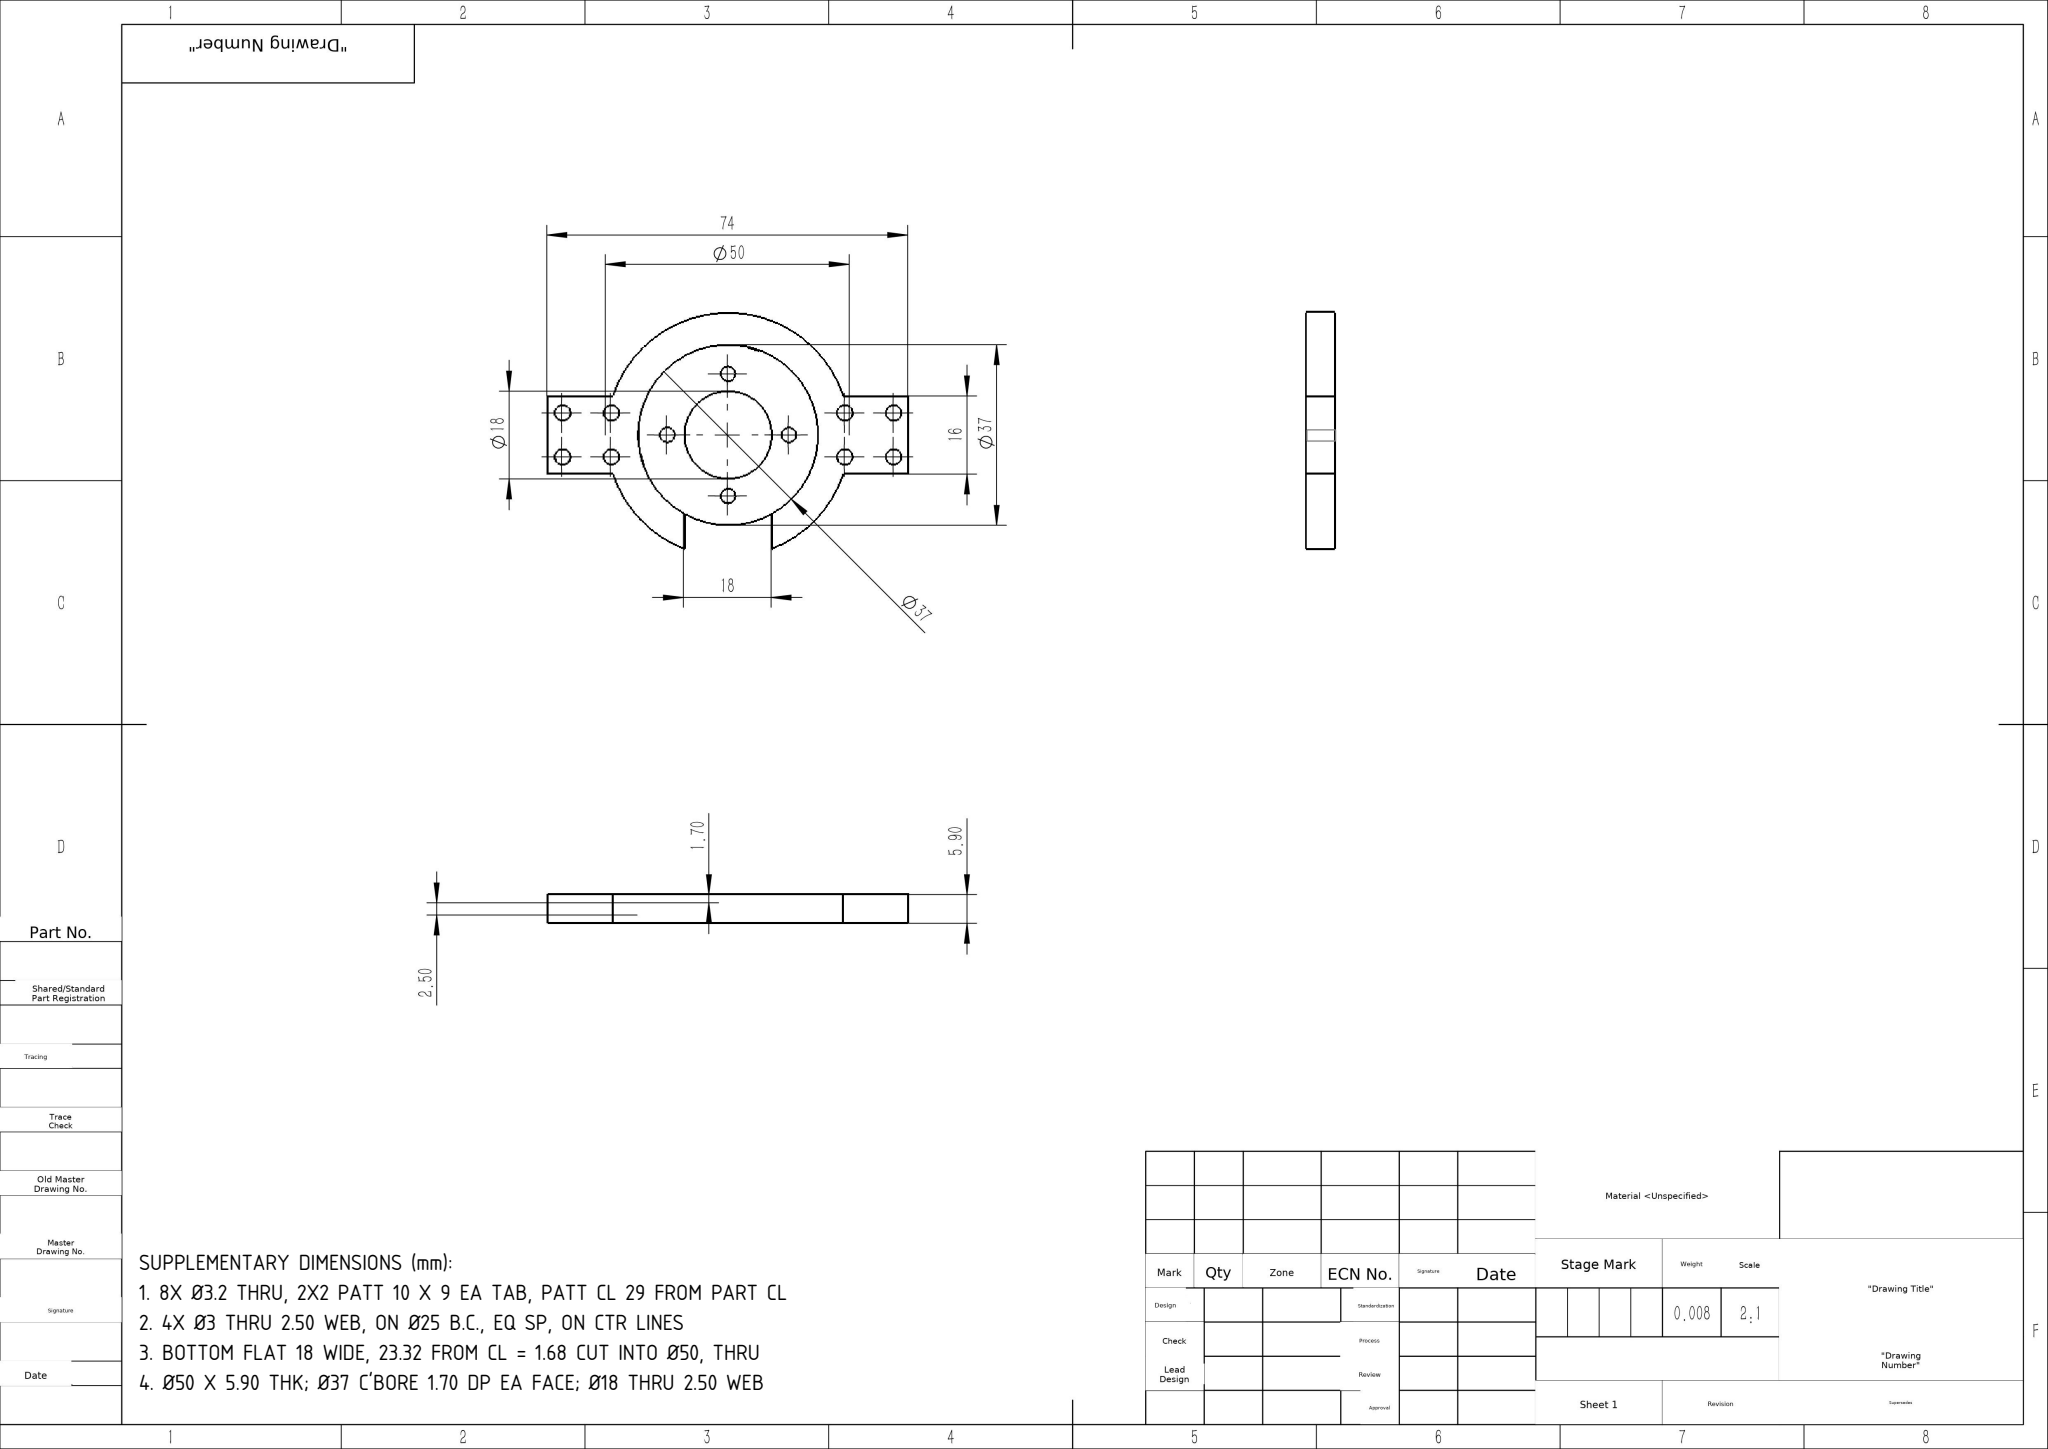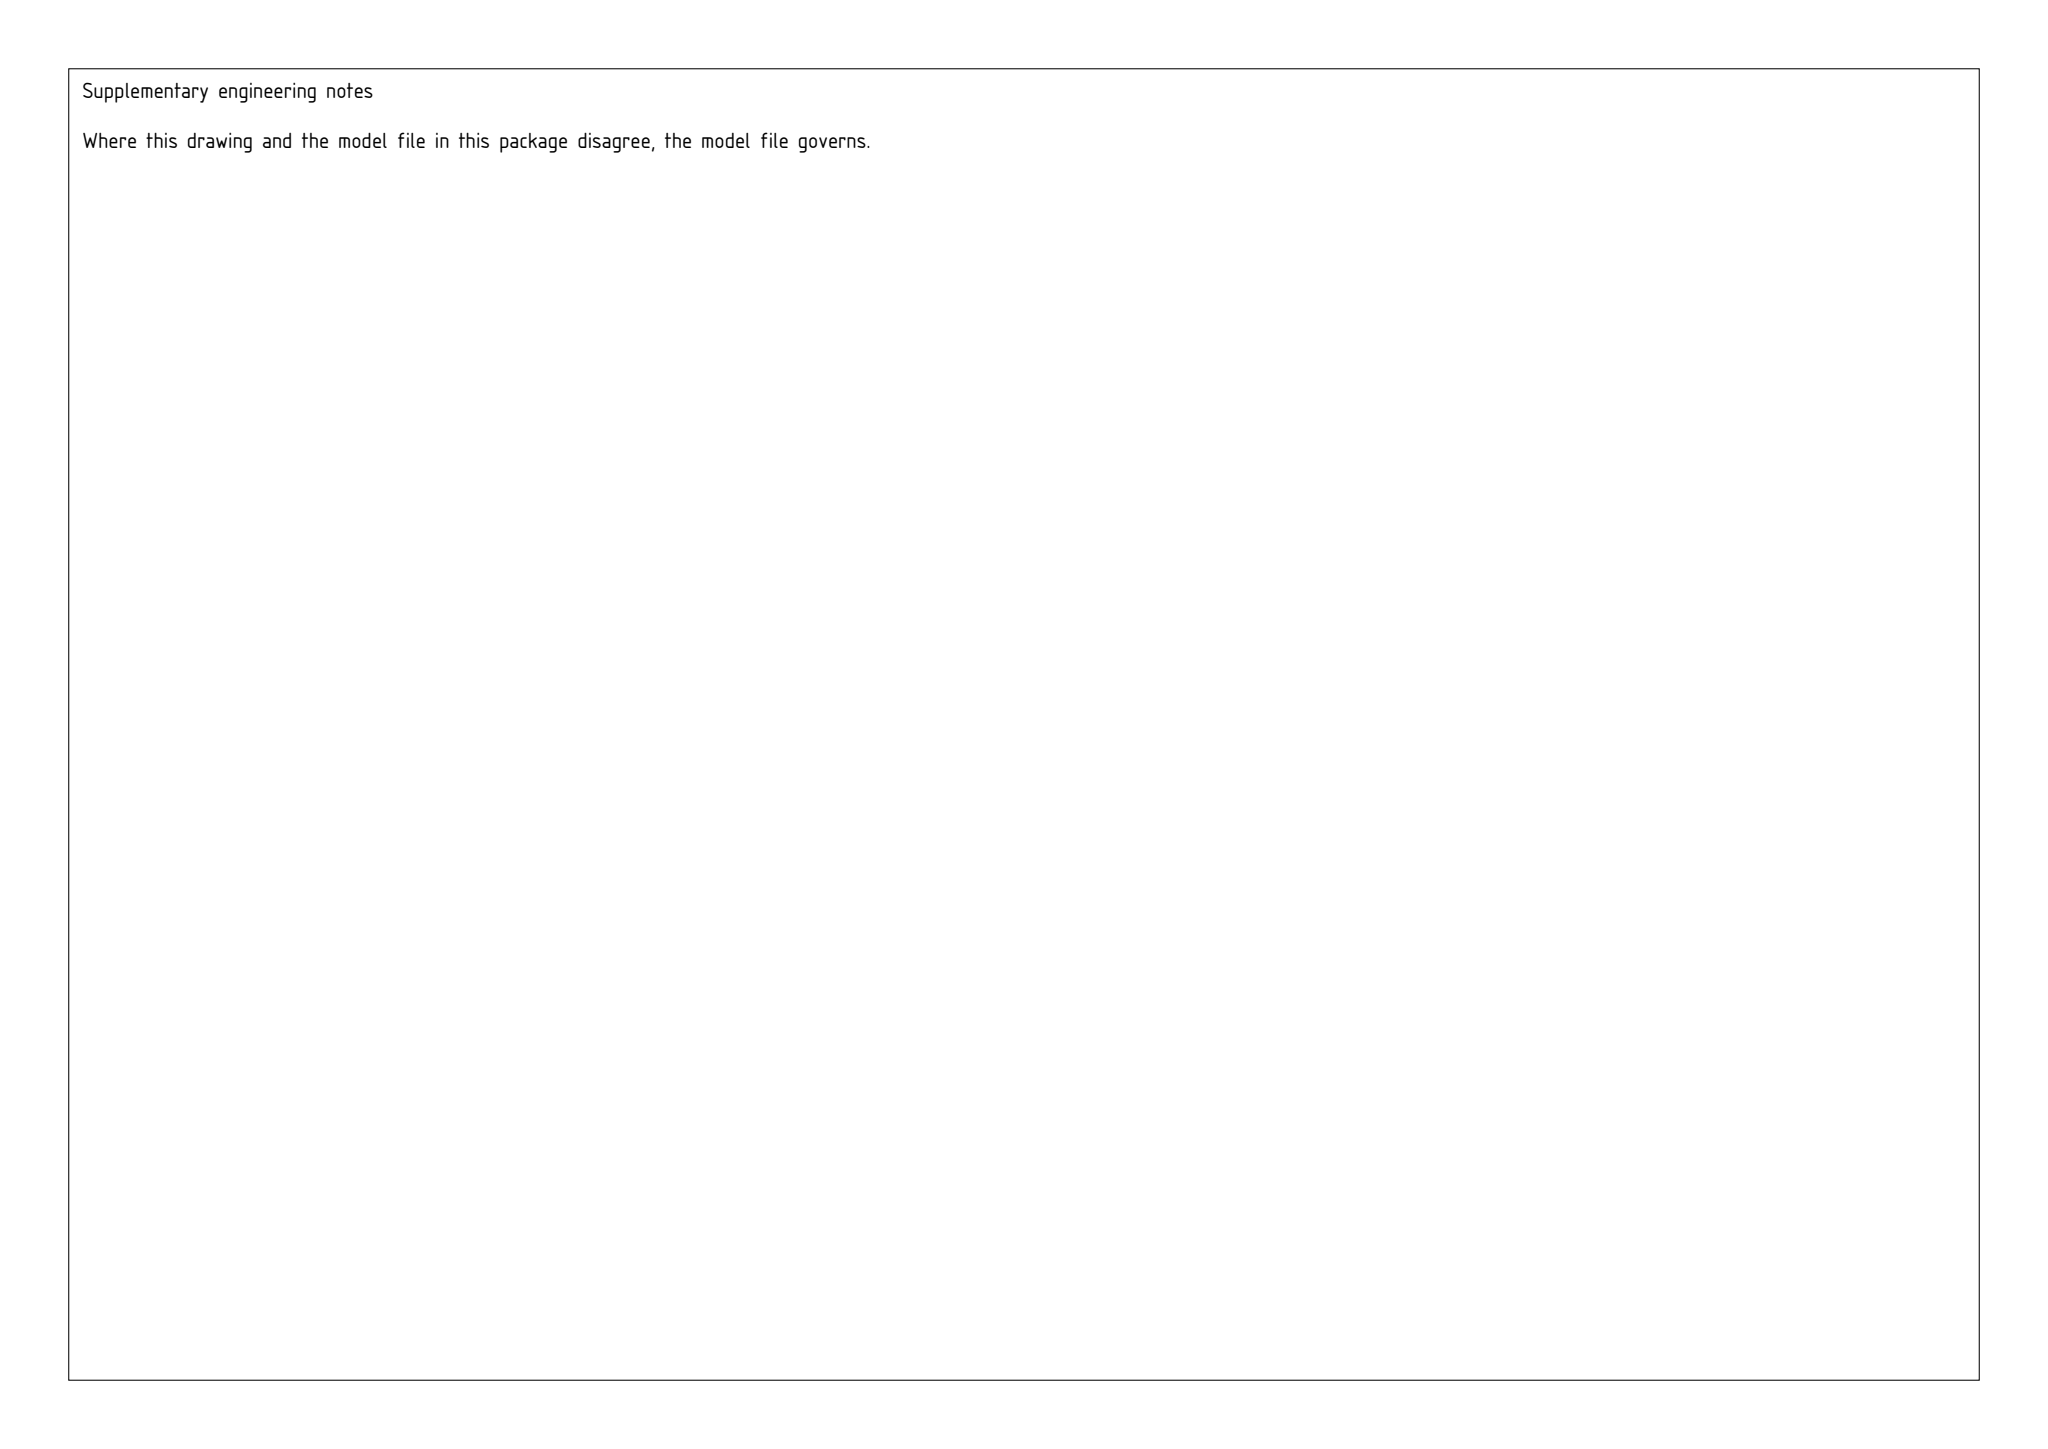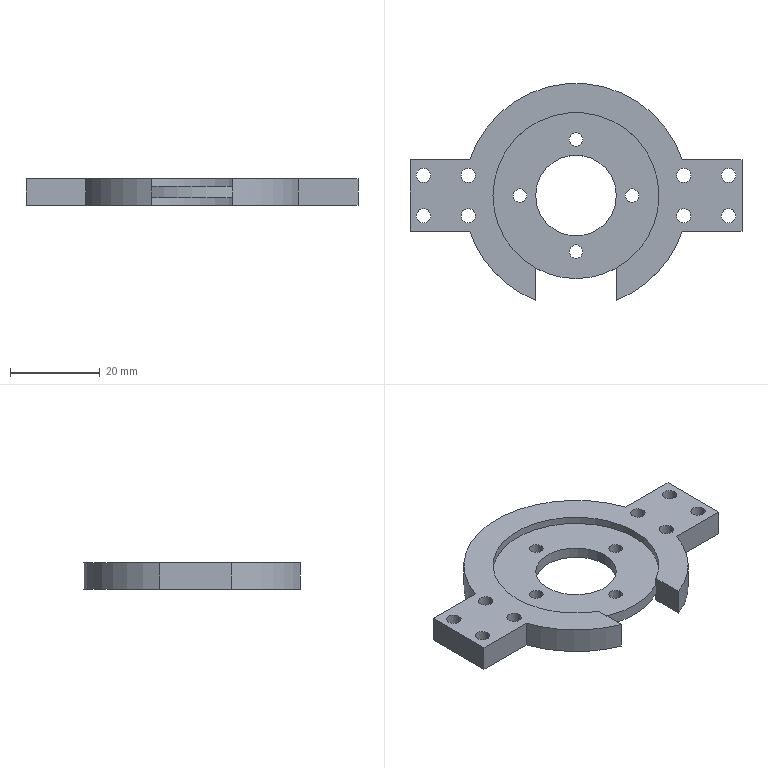Part | SolidWorks | mm | 1 solid | 48 faces | box 74 x 48.32 x 5.9 mm | volume 8478 mm3 | cylinder 36 | plane 12 | commonest cylinder face diameters 3.2 x16 3 x8 37 x7 50 x3 18 x2